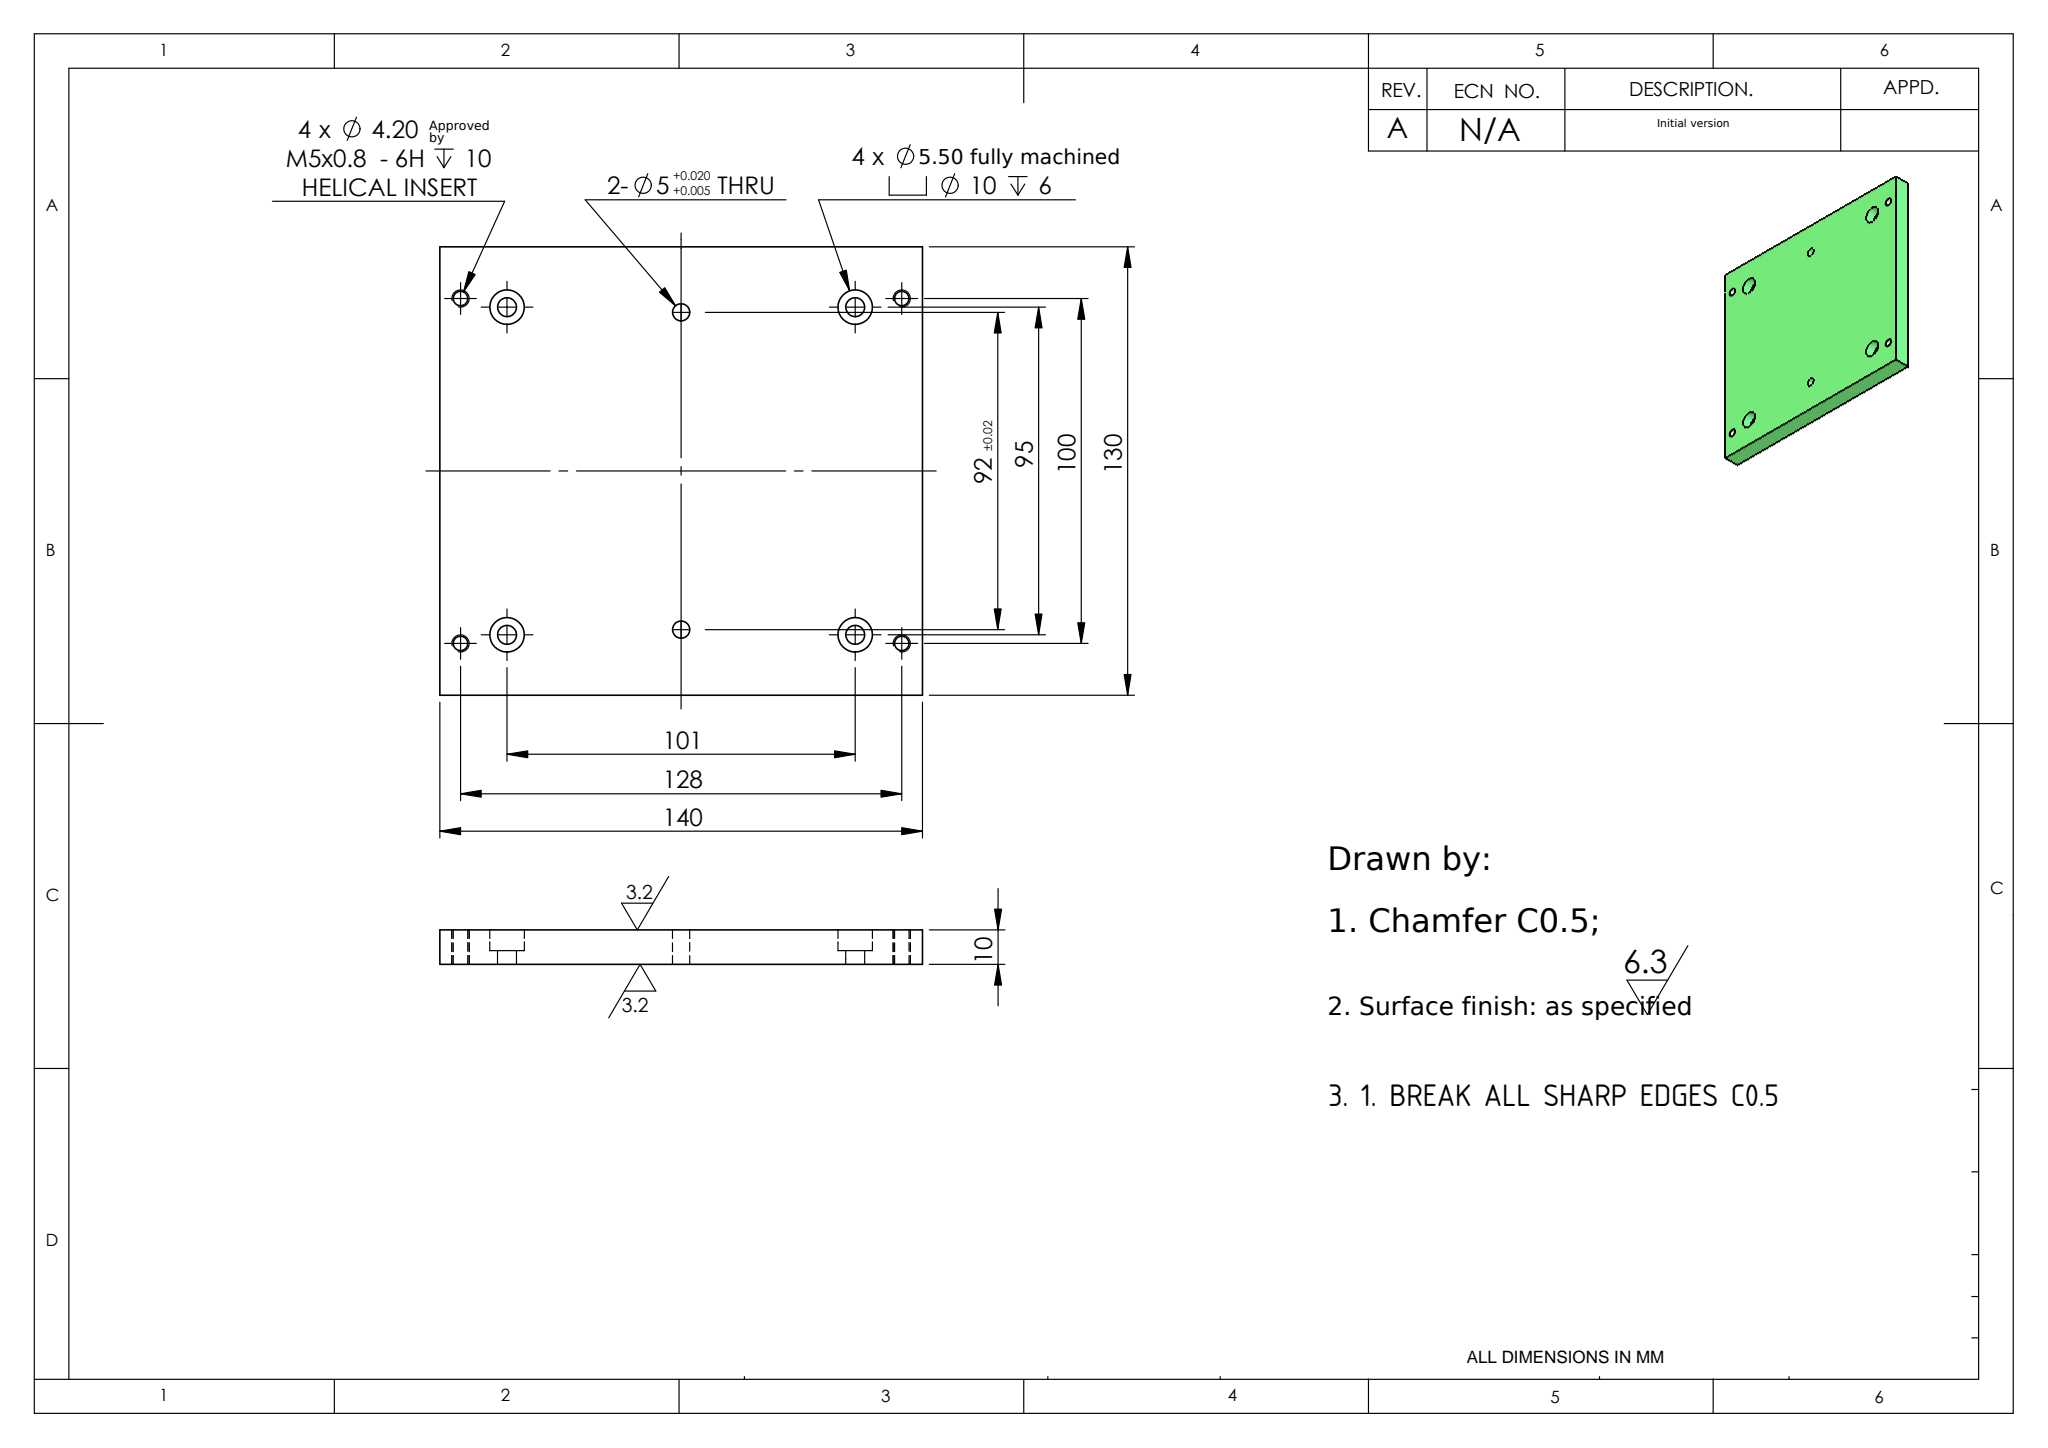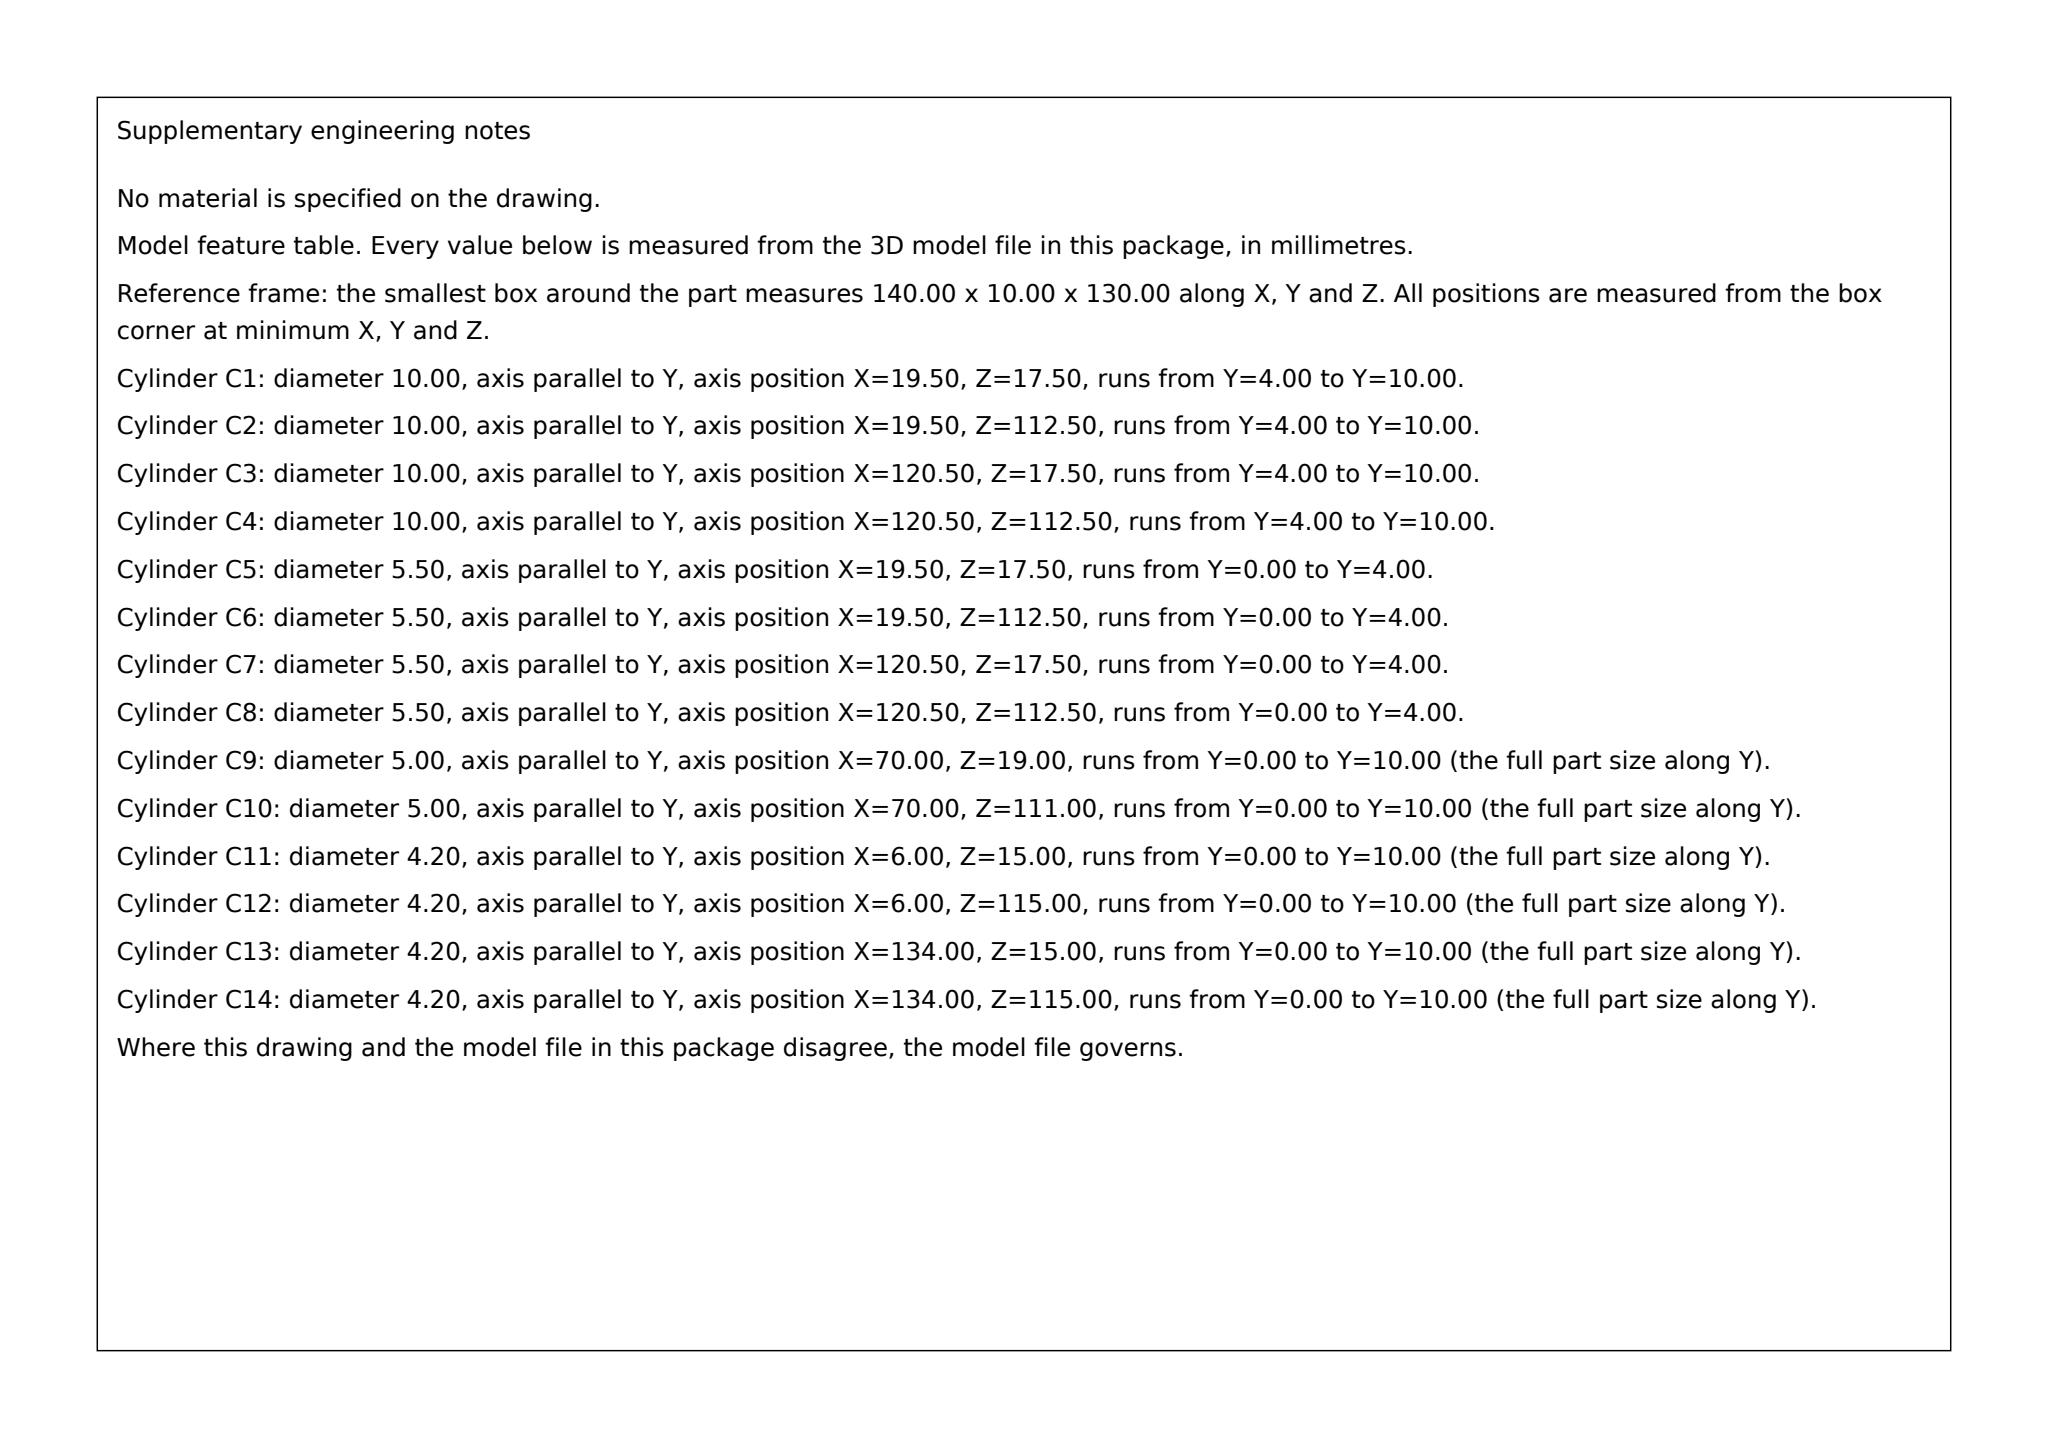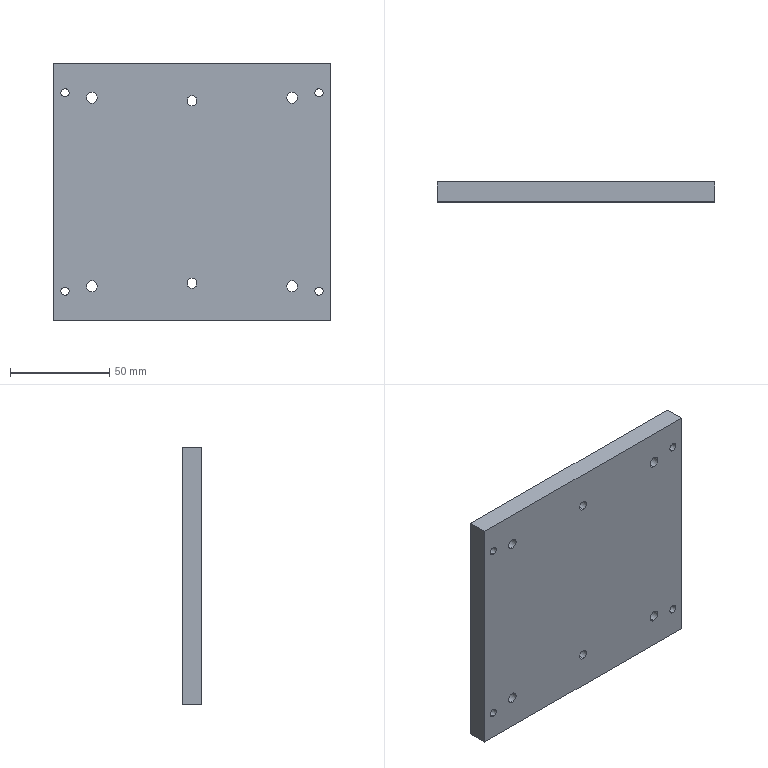Part | SolidWorks | mm | 1 solid | 38 faces | box 140 x 10 x 130 mm | volume 178788 mm3 | cylinder 28 | plane 10 | commonest cylinder face diameters 4.2 x8 5.5 x8 10 x8 5 x4
Drawing notes:
1. BREAK ALL SHARP EDGES C0.5 | from the solid: No fillet radii in STEP; all edges sharp (bbox 140 x 10 x 130), chamfer value C0.5 per note
build123d program:
from build123d import *

# Parameters (mm, degrees)
SKETCH1_W                                            = 140
SKETCH1_H                                            = 130
EXTRUDE1_DEPTH                                       = 10
COUNTERBORE_FOR_M5_HEX_SOCKET_HEAD_CAP_S_D           = 5.5
COUNTERBORE_FOR_M5_HEX_SOCKET_HEAD_CAP_S_CBORE_D     = 10
COUNTERBORE_FOR_M5_HEX_SOCKET_HEAD_CAP_S_CBORE_DEPTH = 6
M5_TAPPED_HOLE_1_D                                   = 4.2
DRILL_1_D                                            = 5


with BuildPart() as part:
    # Sketch1 → Extrude1 (new body)
    with BuildSketch(Plane(origin=(0, 0, 0), x_dir=(1, 0, 0), z_dir=(0, 1, 0))):
        with Locations((70, 65)):
            Rectangle(SKETCH1_W, SKETCH1_H)
    extrude(amount=EXTRUDE1_DEPTH)

    # Counterbore for M5 Hex Socket Head Cap S (through all)
    with Locations(Plane(origin=(0, 10, 0), x_dir=(-1, 0, 0), z_dir=(0, 1, 0))):
        with Locations((-120.5, -112.5), (-19.5, -112.5), (-19.5, -17.5), (-120.5, -17.5)):
            CounterBoreHole(COUNTERBORE_FOR_M5_HEX_SOCKET_HEAD_CAP_S_D / 2, COUNTERBORE_FOR_M5_HEX_SOCKET_HEAD_CAP_S_CBORE_D / 2, COUNTERBORE_FOR_M5_HEX_SOCKET_HEAD_CAP_S_CBORE_DEPTH)

    # M5 Tapped Hole 1 (through all)
    with Locations(Plane(origin=(0, 10, 0), x_dir=(-1, 0, 0), z_dir=(0, 1, 0))):
        with Locations((-134, -115), (-6, -115), (-6, -15), (-134, -15)):
            Hole(M5_TAPPED_HOLE_1_D / 2)

    # Drill 1 (through all)
    with Locations(Plane(origin=(70, 10, -111), x_dir=(0, 0, 1), z_dir=(0, 1, 0))):
        with Locations((0, 0), (92, 0)):
            Hole(DRILL_1_D / 2)


solid = part.part